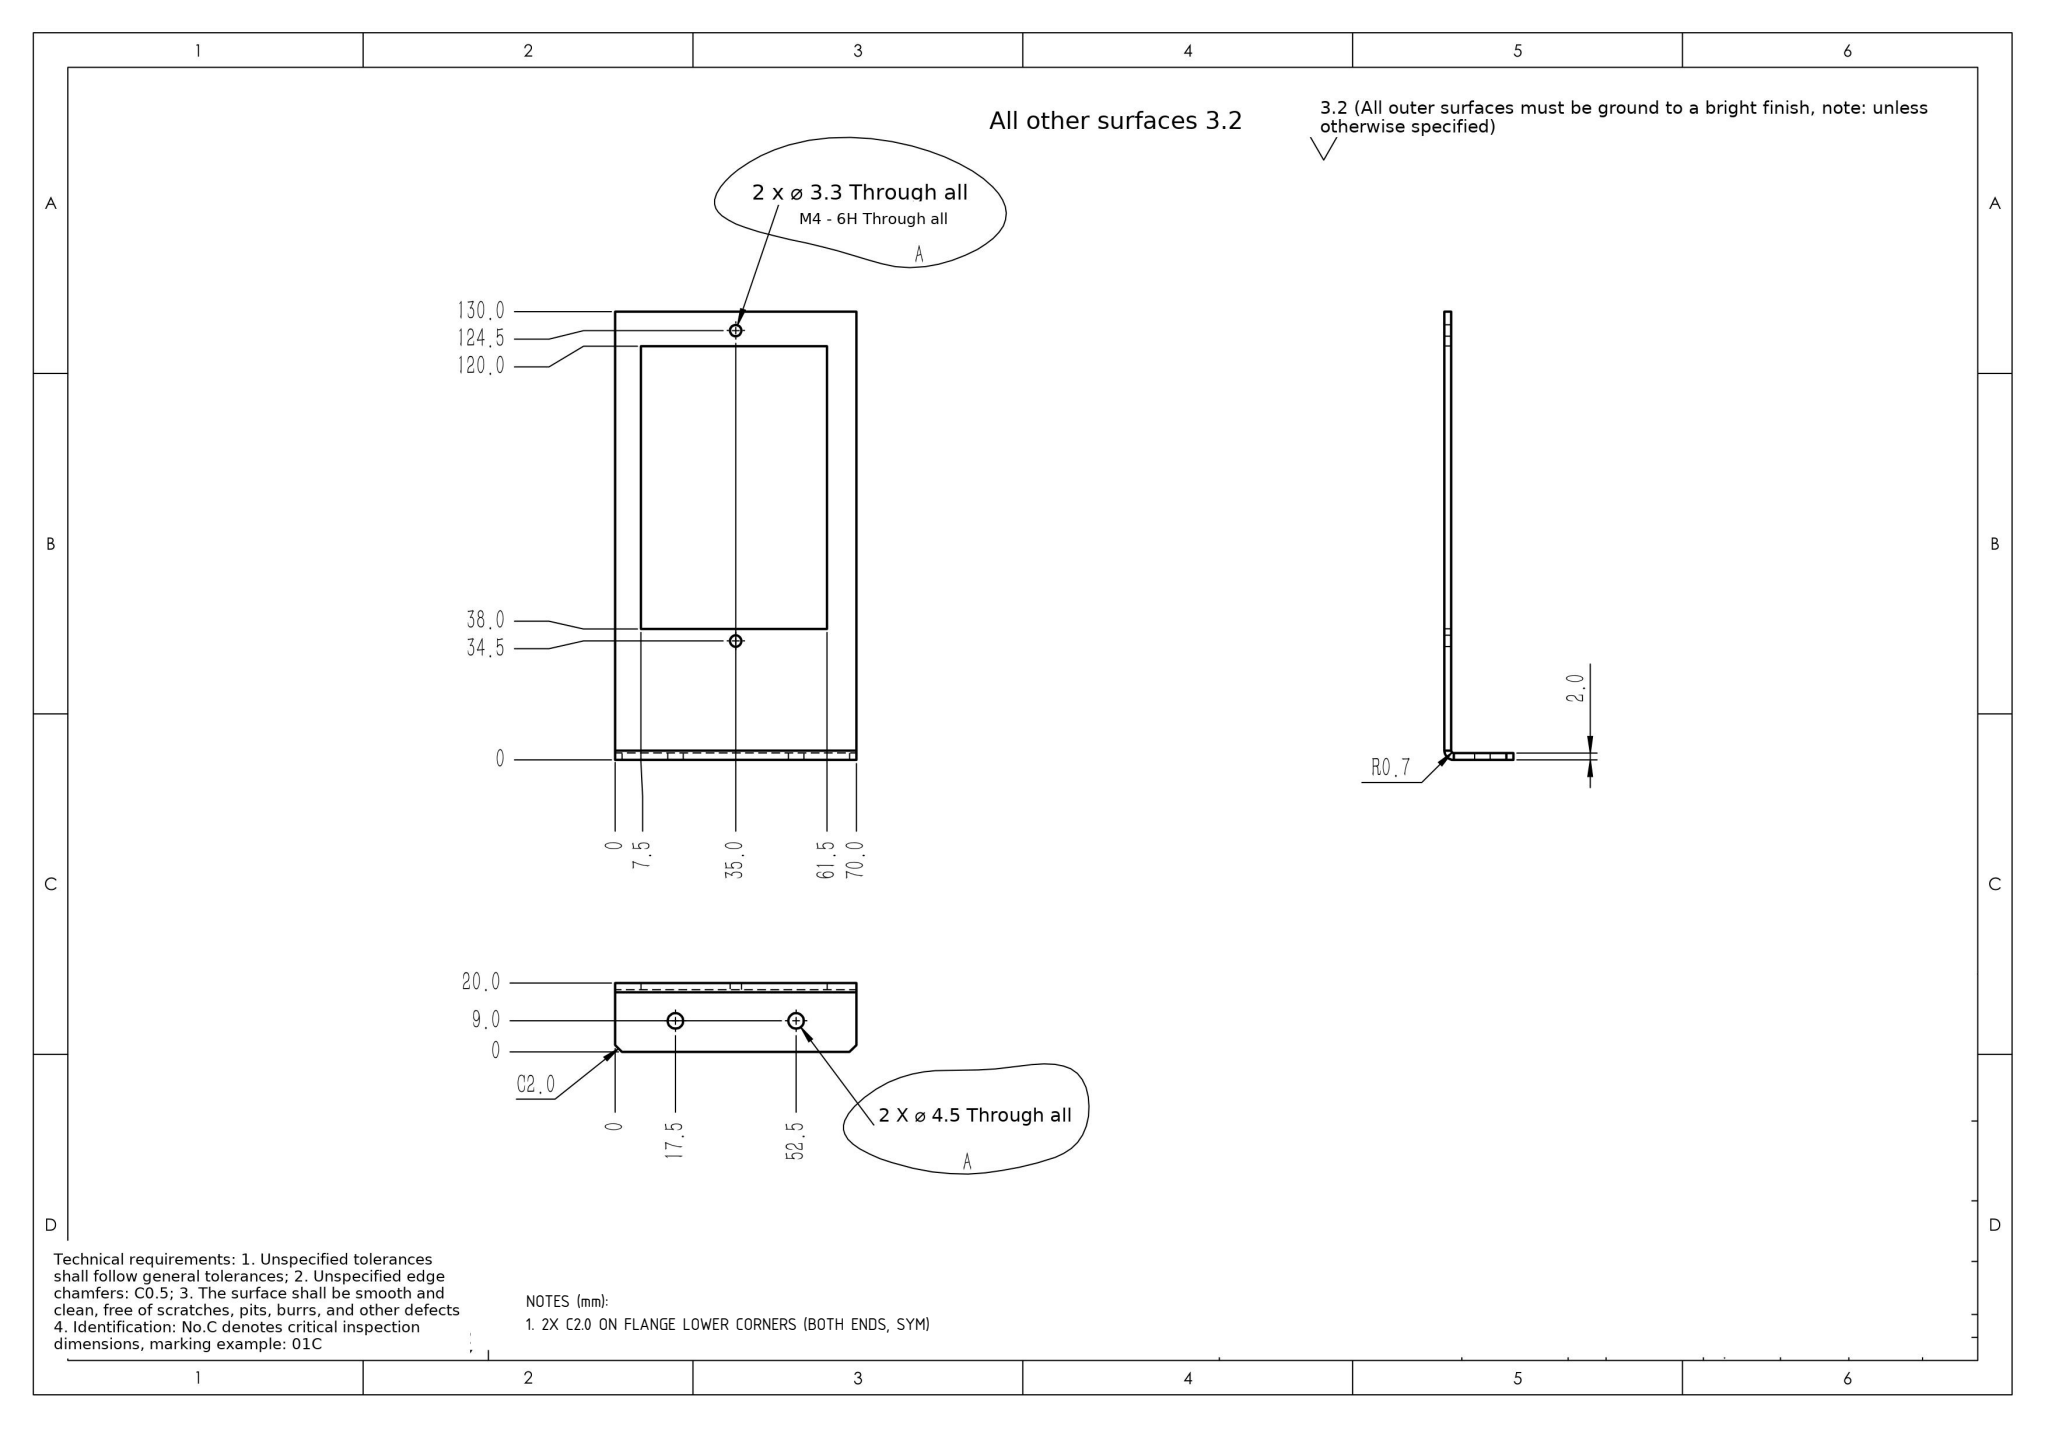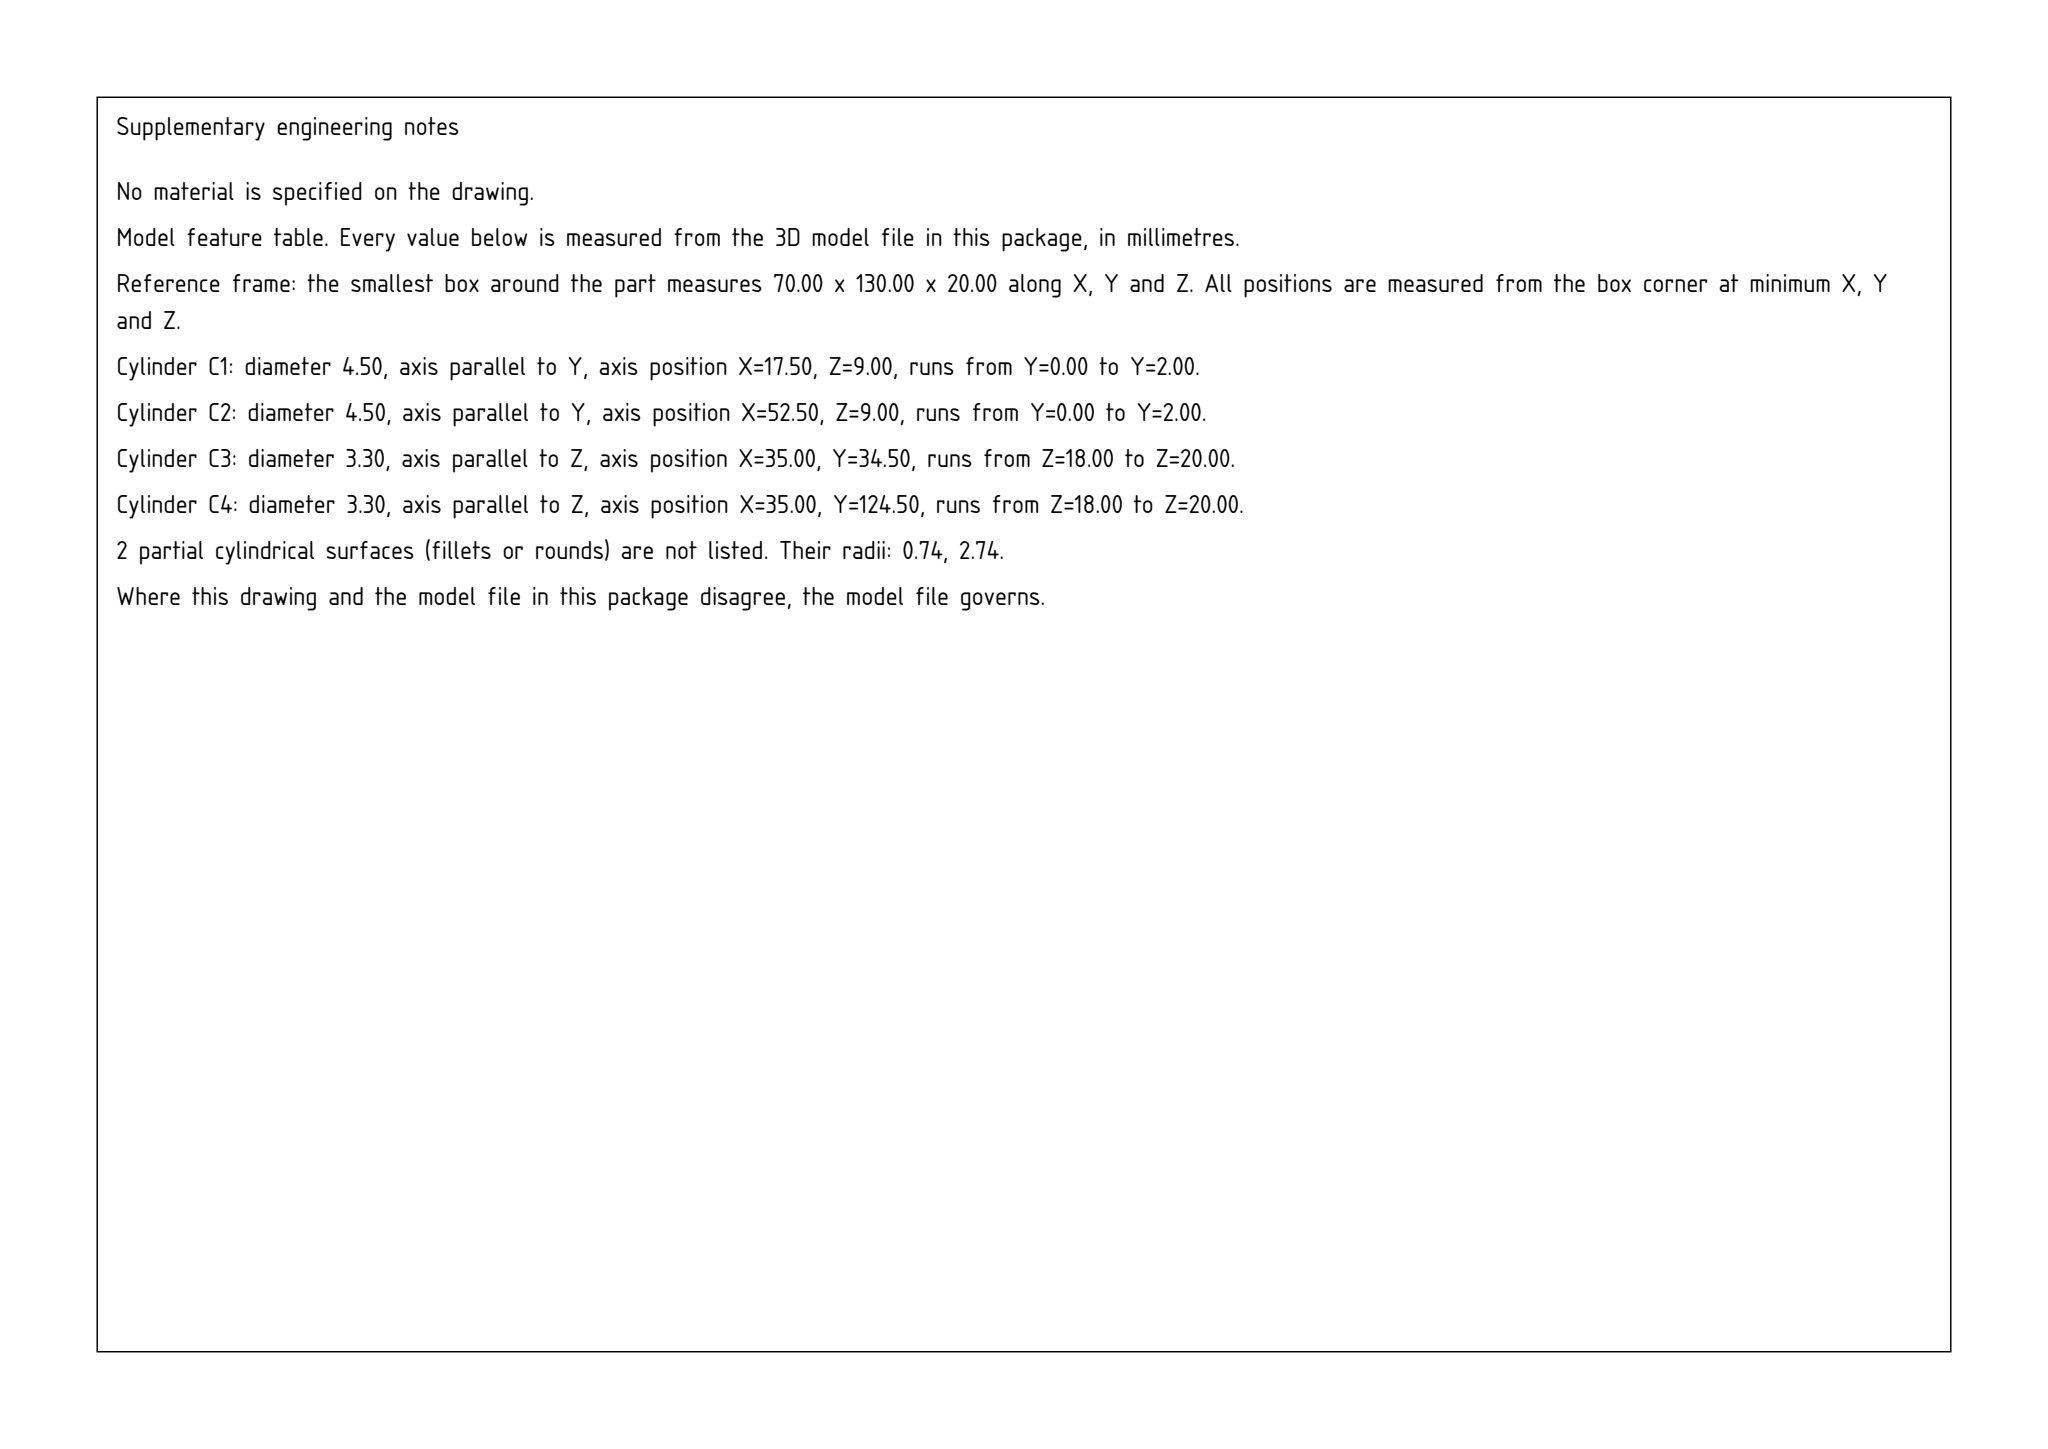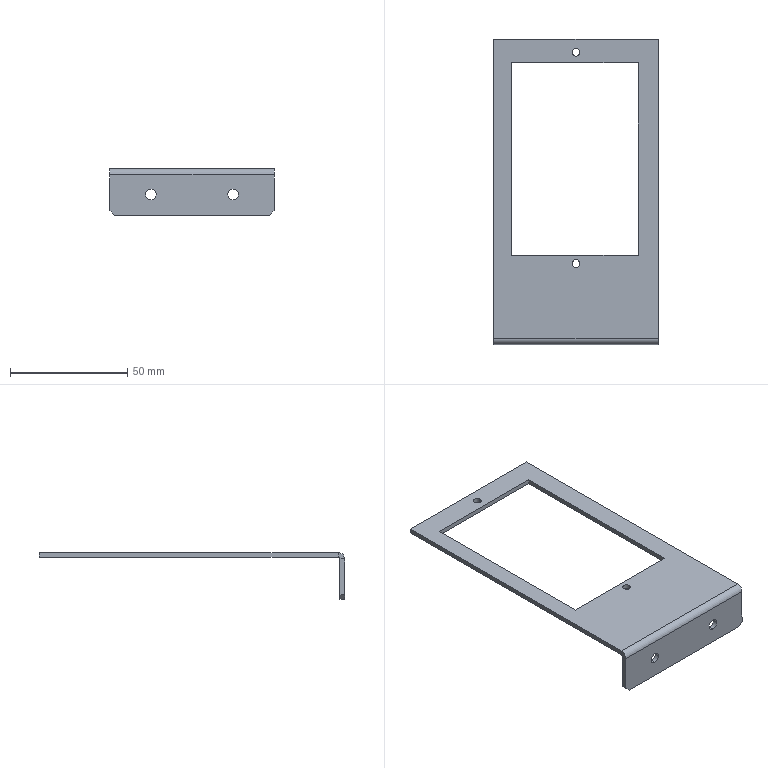Part | SolidWorks | mm | 1 solid | 28 faces | box 70 x 130 x 20 mm | volume 11654 mm3 | plane 18 | cylinder 10 | commonest cylinder face diameters 3.3 x4 4.5 x4 5.473 x1 1.473 x1
Drawing notes:
2X C2.0 ON FLANGE LOWER CORNERS (BOTH ENDS, SYM) | from the solid: x=0 and x=70 each have 3 planes incl. chamfer face; flange 70 long, z 0-20, chamfer 2x2 at both lower corners
STEP:
#1=CARTESIAN_POINT('',(36.65,34.5,0.));
#2=VERTEX_POINT('',#1);
#3=CARTESIAN_POINT('',(33.35,34.5,0.));
#4=VERTEX_POINT('',#3);
#5=CARTESIAN_POINT('',(35.,34.5,0.));
#6=DIRECTION('',(0.,0.,-1.));
#7=DIRECTION('',(-1.,0.,0.));
#8=AXIS2_PLACEMENT_3D('',#5,#6,#7);
#9=CIRCLE('',#8,1.65);
#10=EDGE_CURVE('',#2,#4,#9,.T.);
#11=ORIENTED_EDGE('',*,*,#10,.F.);
#12=CARTESIAN_POINT('',(36.65,34.5,-2.));
#13=VERTEX_POINT('',#12);
#14=CARTESIAN_POINT('',(36.65,34.5,-2.));
#15=DIRECTION('',(0.,0.,-1.));
#16=VECTOR('',#15,1000.);
#17=LINE('',#14,#16);
#18=EDGE_CURVE('',#2,#13,#17,.T.);
#19=ORIENTED_EDGE('',*,*,#18,.T.);
#20=CARTESIAN_POINT('',(33.35,34.5,-2.));
#21=VERTEX_POINT('',#20);
#22=CARTESIAN_POINT('',(35.,34.5,-2.));
#23=DIRECTION('',(0.,0.,-1.));
#24=DIRECTION('',(-1.,0.,0.));
#25=AXIS2_PLACEMENT_3D('',#22,#23,#24);
#26=CIRCLE('',#25,1.65);
#27=EDGE_CURVE('',#13,#21,#26,.T.);
#28=ORIENTED_EDGE('',*,*,#27,.T.);
#29=CARTESIAN_POINT('',(33.35,34.5,-2.));
#30=DIRECTION('',(0.,0.,-1.));
#31=VECTOR('',#30,1000.);
#32=LINE('',#29,#31);
#33=EDGE_CURVE('',#4,#21,#32,.T.);
#34=ORIENTED_EDGE('',*,*,#33,.F.);
#35=EDGE_LOOP('',(#11,#19,#28,#34));
#36=FACE_OUTER_BOUND('',#35,.T.);
#37=CARTESIAN_POINT('',(35.,34.5,-2.));
#38=DIRECTION('',(0.,0.,-1.));
#39=DIRECTION('',(-1.,0.,0.));
#40=AXIS2_PLACEMENT_3D('',#37,#38,#39);
#41=CYLINDRICAL_SURFACE('',#40,1.65);
#42=ADVANCED_FACE('',(#36),#41,.F.);
#43=CARTESIAN_POINT('',(36.65,124.5,0.));
#44=VERTEX_POINT('',#43);
#45=CARTESIAN_POINT('',(33.35,124.5,0.));
#46=VERTEX_POINT('',#45);
#47=CARTESIAN_POINT('',(35.,124.5,0.));
#48=DIRECTION('',(0.,0.,-1.));
#49=DIRECTION('',(-1.,0.,0.));
#50=AXIS2_PLACEMENT_3D('',#47,#48,#49);
#51=CIRCLE('',#50,1.65);
#52=EDGE_CURVE('',#44,#46,#51,.T.);
#53=ORIENTED_EDGE('',*,*,#52,.F.);
#54=CARTESIAN_POINT('',(36.65,124.5,-2.));
#55=VERTEX_POINT('',#54);
#56=CARTESIAN_POINT('',(36.65,124.5,-2.));
#57=DIRECTION('',(0.,0.,-1.));
#58=VECTOR('',#57,1000.);
#59=LINE('',#56,#58);
#60=EDGE_CURVE('',#44,#55,#59,.T.);
#61=ORIENTED_EDGE('',*,*,#60,.T.);
#62=CARTESIAN_POINT('',(33.35,124.5,-2.));
#63=VERTEX_POINT('',#62);
#64=CARTESIAN_POINT('',(35.,124.5,-2.));
#65=DIRECTION('',(0.,0.,-1.));
#66=DIRECTION('',(-1.,0.,0.));
#67=AXIS2_PLACEMENT_3D('',#64,#65,#66);
#68=CIRCLE('',#67,1.65);
#69=EDGE_CURVE('',#55,#63,#68,.T.);
#70=ORIENTED_EDGE('',*,*,#69,.T.);
#71=CARTESIAN_POINT('',(33.35,124.5,-2.));
#72=DIRECTION('',(0.,0.,-1.));
#73=VECTOR('',#72,1000.);
#74=LINE('',#71,#73);
#75=EDGE_CURVE('',#46,#63,#74,.T.);
#76=ORIENTED_EDGE('',*,*,#75,.F.);
#77=EDGE_LOOP('',(#53,#61,#70,#76));
#78=FACE_OUTER_BOUND('',#77,.T.);
#79=CARTESIAN_POINT('',(35.,124.5,-2.));
#80=DIRECTION('',(0.,0.,-1.));
#81=DIRECTION('',(-1.,0.,0.));
#82=AXIS2_PLACEMENT_3D('',#79,#80,#81);
#83=CYLINDRICAL_SURFACE('',#82,1.65);
#84=ADVANCED_FACE('',(#78),#83,.F.);
#85=CARTESIAN_POINT('',(52.5,-0.,-13.25));
#86=VERTEX_POINT('',#85);
#87=CARTESIAN_POINT('',(52.5,-0.,-8.75));
#88=VERTEX_POINT('',#87);
#89=CARTESIAN_POINT('',(52.5,-0.,-11.));
#90=DIRECTION('',(0.,1.,-0.));
#91=DIRECTION('',(0.,0.,1.));
#92=AXIS2_PLACEMENT_3D('',#89,#90,#91);
#93=CIRCLE('',#92,2.25);
#94=EDGE_CURVE('',#86,#88,#93,.T.);
#95=ORIENTED_EDGE('',*,*,#94,.F.);
#96=CARTESIAN_POINT('',(52.5,2.,-13.25));
#97=VERTEX_POINT('',#96);
#98=CARTESIAN_POINT('',(52.5,2.,-13.25));
#99=DIRECTION('',(0.,1.,-0.));
#100=VECTOR('',#99,1000.);
#101=LINE('',#98,#100);
#102=EDGE_CURVE('',#86,#97,#101,.T.);
#103=ORIENTED_EDGE('',*,*,#102,.T.);
#104=CARTESIAN_POINT('',(52.5,2.,-8.75));
#105=VERTEX_POINT('',#104);
#106=CARTESIAN_POINT('',(52.5,2.,-11.));
#107=DIRECTION('',(0.,1.,-0.));
#108=DIRECTION('',(0.,0.,1.));
#109=AXIS2_PLACEMENT_3D('',#106,#107,#108);
#110=CIRCLE('',#109,2.25);
#111=EDGE_CURVE('',#97,#105,#110,.T.);
#112=ORIENTED_EDGE('',*,*,#111,.T.);
#113=CARTESIAN_POINT('',(52.5,2.,-8.75));
#114=DIRECTION('',(0.,1.,-0.));
#115=VECTOR('',#114,1000.);
#116=LINE('',#113,#115);
#117=EDGE_CURVE('',#88,#105,#116,.T.);
#118=ORIENTED_EDGE('',*,*,#117,.F.);
#119=EDGE_LOOP('',(#95,#103,#112,#118));
#120=FACE_OUTER_BOUND('',#119,.T.);
#121=CARTESIAN_POINT('',(52.5,2.,-11.));
#122=DIRECTION('',(0.,1.,-0.));
#123=DIRECTION('',(0.,0.,1.));
#124=AXIS2_PLACEMENT_3D('',#121,#122,#123);
#125=CYLINDRICAL_SURFACE('',#124,2.25);
#126=ADVANCED_FACE('',(#120),#125,.F.);
#127=CARTESIAN_POINT('',(17.5,-0.,-13.25));
#128=VERTEX_POINT('',#127);
#129=CARTESIAN_POINT('',(17.5,-0.,-8.75));
#130=VERTEX_POINT('',#129);
#131=CARTESIAN_POINT('',(17.5,-0.,-11.));
#132=DIRECTION('',(0.,1.,-0.));
#133=DIRECTION('',(0.,0.,1.));
#134=AXIS2_PLACEMENT_3D('',#131,#132,#133);
#135=CIRCLE('',#134,2.25);
#136=EDGE_CURVE('',#128,#130,#135,.T.);
#137=ORIENTED_EDGE('',*,*,#136,.F.);
#138=CARTESIAN_POINT('',(17.5,2.,-13.25));
#139=VERTEX_POINT('',#138);
#140=CARTESIAN_POINT('',(17.5,2.,-13.25));
#141=DIRECTION('',(0.,1.,-0.));
#142=VECTOR('',#141,1000.);
#143=LINE('',#140,#142);
#144=EDGE_CURVE('',#128,#139,#143,.T.);
#145=ORIENTED_EDGE('',*,*,#144,.T.);
#146=CARTESIAN_POINT('',(17.5,2.,-8.75));
#147=VERTEX_POINT('',#146);
#148=CARTESIAN_POINT('',(17.5,2.,-11.));
#149=DIRECTION('',(0.,1.,-0.));
#150=DIRECTION('',(0.,0.,1.));
#151=AXIS2_PLACEMENT_3D('',#148,#149,#150);
#152=CIRCLE('',#151,2.25);
#153=EDGE_CURVE('',#139,#147,#152,.T.);
#154=ORIENTED_EDGE('',*,*,#153,.T.);
#155=CARTESIAN_POINT('',(17.5,2.,-8.75));
#156=DIRECTION('',(0.,1.,-0.));
#157=VECTOR('',#156,1000.);
#158=LINE('',#155,#157);
#159=EDGE_CURVE('',#130,#147,#158,.T.);
#160=ORIENTED_EDGE('',*,*,#159,.F.);
#161=EDGE_LOOP('',(#137,#145,#154,#160));
#162=FACE_OUTER_BOUND('',#161,.T.);
#163=CARTESIAN_POINT('',(17.5,2.,-11.));
#164=DIRECTION('',(0.,1.,-0.));
#165=DIRECTION('',(0.,0.,1.));
#166=AXIS2_PLACEMENT_3D('',#163,#164,#165);
#167=CYLINDRICAL_SURFACE('',#166,2.25);
#168=ADVANCED_FACE('',(#162),#167,.F.);
#169=CARTESIAN_POINT('',(0.,130.,-2.));
#170=VERTEX_POINT('',#169);
#171=CARTESIAN_POINT('',(0.,2.737,-2.));
#172=VERTEX_POINT('',#171);
#173=CARTESIAN_POINT('',(0.,0.,-2.));
#174=DIRECTION('',(0.,-1.,0.));
#175=VECTOR('',#174,1000.);
#176=LINE('',#173,#175);
#177=EDGE_CURVE('',#170,#172,#176,.T.);
#178=ORIENTED_EDGE('',*,*,#177,.T.);
#179=CARTESIAN_POINT('',(0.,2.737,-0.));
#180=VERTEX_POINT('',#179);
#181=CARTESIAN_POINT('',(0.,2.737,-2.));
#182=DIRECTION('',(-0.,0.,1.));
#183=VECTOR('',#182,1000.);
#184=LINE('',#181,#183);
#185=EDGE_CURVE('',#172,#180,#184,.T.);
#186=ORIENTED_EDGE('',*,*,#185,.T.);
#187=CARTESIAN_POINT('',(0.,130.,0.));
#188=VERTEX_POINT('',#187);
#189=CARTESIAN_POINT('',(0.,0.,0.));
#190=DIRECTION('',(0.,-1.,0.));
#191=VECTOR('',#190,1000.);
#192=LINE('',#189,#191);
#193=EDGE_CURVE('',#188,#180,#192,.T.);
#194=ORIENTED_EDGE('',*,*,#193,.F.);
#195=CARTESIAN_POINT('',(0.,130.,-2.));
#196=DIRECTION('',(0.,0.,1.));
#197=VECTOR('',#196,1000.);
#198=LINE('',#195,#197);
#199=EDGE_CURVE('',#170,#188,#198,.T.);
#200=ORIENTED_EDGE('',*,*,#199,.F.);
#201=EDGE_LOOP('',(#178,#186,#194,#200));
#202=FACE_OUTER_BOUND('',#201,.T.);
#203=CARTESIAN_POINT('',(0.,0.,-2.));
#204=DIRECTION('',(-1.,0.,0.));
#205=DIRECTION('',(0.,0.,1.));
#206=AXIS2_PLACEMENT_3D('',#203,#204,#205);
#207=PLANE('',#206);
#208=ADVANCED_FACE('',(#202),#207,.T.);
#209=CARTESIAN_POINT('',(35.,34.5,-2.));
#210=DIRECTION('',(0.,0.,-1.));
#211=DIRECTION('',(-1.,0.,0.));
#212=AXIS2_PLACEMENT_3D('',#209,#210,#211);
#213=CIRCLE('',#212,1.65);
#214=EDGE_CURVE('',#21,#13,#213,.T.);
#215=ORIENTED_EDGE('',*,*,#214,.F.);
#216=ORIENTED_EDGE('',*,*,#27,.F.);
#217=EDGE_LOOP('',(#215,#216));
#218=FACE_BOUND('',#217,.T.);
#219=CARTESIAN_POINT('',(35.,124.5,-2.));
#220=DIRECTION('',(0.,0.,-1.));
#221=DIRECTION('',(-1.,0.,0.));
#222=AXIS2_PLACEMENT_3D('',#219,#220,#221);
#223=CIRCLE('',#222,1.65);
#224=EDGE_CURVE('',#63,#55,#223,.T.);
#225=ORIENTED_EDGE('',*,*,#224,.F.);
#226=ORIENTED_EDGE('',*,*,#69,.F.);
#227=EDGE_LOOP('',(#225,#226));
#228=FACE_BOUND('',#227,.T.);
#229=CARTESIAN_POINT('',(7.5,38.,-2.));
#230=VERTEX_POINT('',#229);
#231=CARTESIAN_POINT('',(7.5,120.,-2.));
#232=VERTEX_POINT('',#231);
#233=CARTESIAN_POINT('',(7.5,120.,-2.));
#234=DIRECTION('',(0.,1.,0.));
#235=VECTOR('',#234,1000.);
#236=LINE('',#233,#235);
#237=EDGE_CURVE('',#230,#232,#236,.T.);
#238=ORIENTED_EDGE('',*,*,#237,.F.);
#239=CARTESIAN_POINT('',(61.5,38.,-2.));
#240=VERTEX_POINT('',#239);
#241=CARTESIAN_POINT('',(7.5,38.,-2.));
#242=DIRECTION('',(-1.,0.,0.));
#243=VECTOR('',#242,1000.);
#244=LINE('',#241,#243);
#245=EDGE_CURVE('',#240,#230,#244,.T.);
#246=ORIENTED_EDGE('',*,*,#245,.F.);
#247=CARTESIAN_POINT('',(61.5,120.,-2.));
#248=VERTEX_POINT('',#247);
#249=CARTESIAN_POINT('',(61.5,120.,-2.));
#250=DIRECTION('',(0.,-1.,0.));
#251=VECTOR('',#250,1000.);
#252=LINE('',#249,#251);
#253=EDGE_CURVE('',#248,#240,#252,.T.);
#254=ORIENTED_EDGE('',*,*,#253,.F.);
#255=CARTESIAN_POINT('',(7.5,120.,-2.));
#256=DIRECTION('',(1.,0.,0.));
#257=VECTOR('',#256,1000.);
#258=LINE('',#255,#257);
#259=EDGE_CURVE('',#232,#248,#258,.T.);
#260=ORIENTED_EDGE('',*,*,#259,.F.);
#261=EDGE_LOOP('',(#238,#246,#254,#260));
#262=FACE_BOUND('',#261,.T.);
#263=CARTESIAN_POINT('',(70.,2.737,-2.));
#264=VERTEX_POINT('',#263);
#265=CARTESIAN_POINT('',(70.,130.,-2.));
#266=VERTEX_POINT('',#265);
#267=CARTESIAN_POINT('',(70.,0.,-2.));
#268=DIRECTION('',(0.,1.,0.));
#269=VECTOR('',#268,1000.);
#270=LINE('',#267,#269);
#271=EDGE_CURVE('',#264,#266,#270,.T.);
#272=ORIENTED_EDGE('',*,*,#271,.F.);
#273=CARTESIAN_POINT('',(0.,2.737,-2.));
#274=DIRECTION('',(1.,0.,0.));
#275=VECTOR('',#274,1000.);
#276=LINE('',#273,#275);
#277=EDGE_CURVE('',#172,#264,#276,.T.);
#278=ORIENTED_EDGE('',*,*,#277,.F.);
#279=ORIENTED_EDGE('',*,*,#177,.F.);
#280=CARTESIAN_POINT('',(0.,130.,-2.));
#281=DIRECTION('',(-1.,0.,0.));
#282=VECTOR('',#281,1000.);
#283=LINE('',#280,#282);
#284=EDGE_CURVE('',#266,#170,#283,.T.);
#285=ORIENTED_EDGE('',*,*,#284,.F.);
#286=EDGE_LOOP('',(#272,#278,#279,#285));
#287=FACE_OUTER_BOUND('',#286,.T.);
#288=CARTESIAN_POINT('',(0.,0.,-2.));
#289=DIRECTION('',(0.,0.,-1.));
#290=DIRECTION('',(-1.,0.,0.));
#291=AXIS2_PLACEMENT_3D('',#288,#289,#290);
#292=PLANE('',#291);
#293=ADVANCED_FACE('',(#218,#228,#262,#287),#292,.T.);
#294=CARTESIAN_POINT('',(35.,34.5,0.));
#295=DIRECTION('',(0.,0.,-1.));
#296=DIRECTION('',(-1.,0.,0.));
#297=AXIS2_PLACEMENT_3D('',#294,#295,#296);
#298=CIRCLE('',#297,1.65);
#299=EDGE_CURVE('',#4,#2,#298,.T.);
#300=ORIENTED_EDGE('',*,*,#299,.T.);
#301=ORIENTED_EDGE('',*,*,#10,.T.);
#302=EDGE_LOOP('',(#300,#301));
#303=FACE_BOUND('',#302,.T.);
#304=CARTESIAN_POINT('',(35.,124.5,0.));
#305=DIRECTION('',(0.,0.,-1.));
#306=DIRECTION('',(-1.,0.,0.));
#307=AXIS2_PLACEMENT_3D('',#304,#305,#306);
#308=CIRCLE('',#307,1.65);
#309=EDGE_CURVE('',#46,#44,#308,.T.);
#310=ORIENTED_EDGE('',*,*,#309,.T.);
#311=ORIENTED_EDGE('',*,*,#52,.T.);
#312=EDGE_LOOP('',(#310,#311));
#313=FACE_BOUND('',#312,.T.);
#314=CARTESIAN_POINT('',(61.5,38.,0.));
#315=VERTEX_POINT('',#314);
#316=CARTESIAN_POINT('',(7.5,38.,0.));
#317=VERTEX_POINT('',#316);
#318=CARTESIAN_POINT('',(0.,38.,0.));
#319=DIRECTION('',(-1.,0.,0.));
#320=VECTOR('',#319,1000.);
#321=LINE('',#318,#320);
#322=EDGE_CURVE('',#315,#317,#321,.T.);
#323=ORIENTED_EDGE('',*,*,#322,.T.);
#324=CARTESIAN_POINT('',(7.5,120.,0.));
#325=VERTEX_POINT('',#324);
#326=CARTESIAN_POINT('',(7.5,-0.,0.));
#327=DIRECTION('',(0.,1.,0.));
#328=VECTOR('',#327,1000.);
#329=LINE('',#326,#328);
#330=EDGE_CURVE('',#317,#325,#329,.T.);
#331=ORIENTED_EDGE('',*,*,#330,.T.);
#332=CARTESIAN_POINT('',(61.5,120.,0.));
#333=VERTEX_POINT('',#332);
#334=CARTESIAN_POINT('',(0.,120.,0.));
#335=DIRECTION('',(1.,0.,0.));
#336=VECTOR('',#335,1000.);
#337=LINE('',#334,#336);
#338=EDGE_CURVE('',#325,#333,#337,.T.);
#339=ORIENTED_EDGE('',*,*,#338,.T.);
#340=CARTESIAN_POINT('',(61.5,0.,0.));
#341=DIRECTION('',(0.,-1.,0.));
#342=VECTOR('',#341,1000.);
#343=LINE('',#340,#342);
#344=EDGE_CURVE('',#333,#315,#343,.T.);
#345=ORIENTED_EDGE('',*,*,#344,.T.);
#346=EDGE_LOOP('',(#323,#331,#339,#345));
#347=FACE_BOUND('',#346,.T.);
#348=CARTESIAN_POINT('',(70.,2.737,0.));
#349=VERTEX_POINT('',#348);
#350=CARTESIAN_POINT('',(0.,2.737,-0.));
#351=DIRECTION('',(1.,0.,0.));
#352=VECTOR('',#351,1000.);
#353=LINE('',#350,#352);
#354=EDGE_CURVE('',#180,#349,#353,.T.);
#355=ORIENTED_EDGE('',*,*,#354,.T.);
#356=CARTESIAN_POINT('',(70.,130.,0.));
#357=VERTEX_POINT('',#356);
#358=CARTESIAN_POINT('',(70.,0.,0.));
#359=DIRECTION('',(0.,1.,0.));
#360=VECTOR('',#359,1000.);
#361=LINE('',#358,#360);
#362=EDGE_CURVE('',#349,#357,#361,.T.);
#363=ORIENTED_EDGE('',*,*,#362,.T.);
#364=CARTESIAN_POINT('',(0.,130.,0.));
#365=DIRECTION('',(-1.,0.,0.));
#366=VECTOR('',#365,1000.);
#367=LINE('',#364,#366);
#368=EDGE_CURVE('',#357,#188,#367,.T.);
#369=ORIENTED_EDGE('',*,*,#368,.T.);
#370=ORIENTED_EDGE('',*,*,#193,.T.);
#371=EDGE_LOOP('',(#355,#363,#369,#370));
#372=FACE_OUTER_BOUND('',#371,.T.);
#373=CARTESIAN_POINT('',(0.,0.,0.));
#374=DIRECTION('',(0.,0.,-1.));
#375=DIRECTION('',(-1.,0.,0.));
#376=AXIS2_PLACEMENT_3D('',#373,#374,#375);
#377=PLANE('',#376);
#378=ADVANCED_FACE('',(#303,#313,#347,#372),#377,.F.);
#379=ORIENTED_EDGE('',*,*,#368,.F.);
#380=CARTESIAN_POINT('',(70.,130.,-2.));
#381=DIRECTION('',(0.,0.,1.));
#382=VECTOR('',#381,1000.);
#383=LINE('',#380,#382);
#384=EDGE_CURVE('',#266,#357,#383,.T.);
#385=ORIENTED_EDGE('',*,*,#384,.F.);
#386=ORIENTED_EDGE('',*,*,#284,.T.);
#387=ORIENTED_EDGE('',*,*,#199,.T.);
#388=EDGE_LOOP('',(#379,#385,#386,#387));
#389=FACE_OUTER_BOUND('',#388,.T.);
#390=CARTESIAN_POINT('',(0.,130.,-2.));
#391=DIRECTION('',(0.,1.,0.));
#392=DIRECTION('',(0.,0.,1.));
#393=AXIS2_PLACEMENT_3D('',#390,#391,#392);
#394=PLANE('',#393);
#395=ADVANCED_FACE('',(#389),#394,.T.);
#396=CARTESIAN_POINT('',(70.,2.737,-2.));
#397=DIRECTION('',(0.,0.,1.));
#398=VECTOR('',#397,1000.);
#399=LINE('',#396,#398);
#400=EDGE_CURVE('',#264,#349,#399,.T.);
#401=ORIENTED_EDGE('',*,*,#400,.F.);
#402=ORIENTED_EDGE('',*,*,#271,.T.);
#403=ORIENTED_EDGE('',*,*,#384,.T.);
#404=ORIENTED_EDGE('',*,*,#362,.F.);
#405=EDGE_LOOP('',(#401,#402,#403,#404));
#406=FACE_OUTER_BOUND('',#405,.T.);
#407=CARTESIAN_POINT('',(70.,0.,-2.));
#408=DIRECTION('',(1.,0.,0.));
#409=DIRECTION('',(0.,0.,-1.));
#410=AXIS2_PLACEMENT_3D('',#407,#408,#409);
#411=PLANE('',#410);
#412=ADVANCED_FACE('',(#406),#411,.T.);
#413=CARTESIAN_POINT('',(70.,2.,-2.737));
#414=VERTEX_POINT('',#413);
#415=CARTESIAN_POINT('',(70.,-0.,-2.737));
#416=VERTEX_POINT('',#415);
#417=CARTESIAN_POINT('',(70.,-0.,-2.737));
#418=DIRECTION('',(0.,-1.,0.));
#419=VECTOR('',#418,1000.);
#420=LINE('',#417,#419);
#421=EDGE_CURVE('',#414,#416,#420,.T.);
#422=ORIENTED_EDGE('',*,*,#421,.F.);
#423=CARTESIAN_POINT('',(70.,2.737,-2.737));
#424=DIRECTION('',(1.,0.,0.));
#425=DIRECTION('',(0.,0.,1.));
#426=AXIS2_PLACEMENT_3D('',#423,#424,#425);
#427=CIRCLE('',#426,0.7366);
#428=EDGE_CURVE('',#264,#414,#427,.T.);
#429=ORIENTED_EDGE('',*,*,#428,.F.);
#430=ORIENTED_EDGE('',*,*,#400,.T.);
#431=CARTESIAN_POINT('',(70.,2.737,-2.737));
#432=DIRECTION('',(1.,0.,0.));
#433=DIRECTION('',(0.,0.,1.));
#434=AXIS2_PLACEMENT_3D('',#431,#432,#433);
#435=CIRCLE('',#434,2.737);
#436=EDGE_CURVE('',#349,#416,#435,.T.);
#437=ORIENTED_EDGE('',*,*,#436,.T.);
#438=EDGE_LOOP('',(#422,#429,#430,#437));
#439=FACE_OUTER_BOUND('',#438,.T.);
#440=CARTESIAN_POINT('',(70.,2.737,-2.737));
#441=DIRECTION('',(1.,0.,0.));
#442=DIRECTION('',(0.,0.,-1.));
#443=AXIS2_PLACEMENT_3D('',#440,#441,#442);
#444=PLANE('',#443);
#445=ADVANCED_FACE('',(#439),#444,.T.);
#446=CARTESIAN_POINT('',(0.,2.,-2.737));
#447=VERTEX_POINT('',#446);
#448=CARTESIAN_POINT('',(0.,2.737,-2.737));
#449=DIRECTION('',(-1.,0.,0.));
#450=DIRECTION('',(0.,0.,1.));
#451=AXIS2_PLACEMENT_3D('',#448,#449,#450);
#452=CIRCLE('',#451,0.7366);
#453=EDGE_CURVE('',#447,#172,#452,.T.);
#454=ORIENTED_EDGE('',*,*,#453,.F.);
#455=CARTESIAN_POINT('',(0.,-0.,-2.737));
#456=VERTEX_POINT('',#455);
#457=CARTESIAN_POINT('',(0.,2.,-2.737));
#458=DIRECTION('',(0.,-1.,0.));
#459=VECTOR('',#458,1000.);
#460=LINE('',#457,#459);
#461=EDGE_CURVE('',#447,#456,#460,.T.);
#462=ORIENTED_EDGE('',*,*,#461,.T.);
#463=CARTESIAN_POINT('',(0.,2.737,-2.737));
#464=DIRECTION('',(-1.,0.,0.));
#465=DIRECTION('',(0.,0.,1.));
#466=AXIS2_PLACEMENT_3D('',#463,#464,#465);
#467=CIRCLE('',#466,2.737);
#468=EDGE_CURVE('',#456,#180,#467,.T.);
#469=ORIENTED_EDGE('',*,*,#468,.T.);
#470=ORIENTED_EDGE('',*,*,#185,.F.);
#471=EDGE_LOOP('',(#454,#462,#469,#470));
#472=FACE_OUTER_BOUND('',#471,.T.);
#473=CARTESIAN_POINT('',(0.,2.737,-2.737));
#474=DIRECTION('',(1.,0.,0.));
#475=DIRECTION('',(0.,0.,-1.));
#476=AXIS2_PLACEMENT_3D('',#473,#474,#475);
#477=PLANE('',#476);
#478=ADVANCED_FACE('',(#472),#477,.F.);
#479=ORIENTED_EDGE('',*,*,#354,.F.);
#480=ORIENTED_EDGE('',*,*,#468,.F.);
#481=CARTESIAN_POINT('',(70.,-0.,-2.737));
#482=DIRECTION('',(1.,0.,0.));
#483=VECTOR('',#482,1000.);
#484=LINE('',#481,#483);
#485=EDGE_CURVE('',#456,#416,#484,.T.);
#486=ORIENTED_EDGE('',*,*,#485,.T.);
#487=ORIENTED_EDGE('',*,*,#436,.F.);
#488=EDGE_LOOP('',(#479,#480,#486,#487));
#489=FACE_OUTER_BOUND('',#488,.T.);
#490=CARTESIAN_POINT('',(0.,2.737,-2.737));
#491=DIRECTION('',(-1.,0.,0.));
#492=DIRECTION('',(0.,-1.,0.));
#493=AXIS2_PLACEMENT_3D('',#490,#491,#492);
#494=CYLINDRICAL_SURFACE('',#493,2.737);
#495=ADVANCED_FACE('',(#489),#494,.T.);
#496=ORIENTED_EDGE('',*,*,#277,.T.);
#497=ORIENTED_EDGE('',*,*,#428,.T.);
#498=CARTESIAN_POINT('',(70.,2.,-2.737));
#499=DIRECTION('',(-1.,0.,0.));
#500=VECTOR('',#499,1000.);
#501=LINE('',#498,#500);
#502=EDGE_CURVE('',#414,#447,#501,.T.);
#503=ORIENTED_EDGE('',*,*,#502,.T.);
#504=ORIENTED_EDGE('',*,*,#453,.T.);
#505=EDGE_LOOP('',(#496,#497,#503,#504));
#506=FACE_OUTER_BOUND('',#505,.T.);
#507=CARTESIAN_POINT('',(0.,2.737,-2.737));
#508=DIRECTION('',(-1.,0.,0.));
#509=DIRECTION('',(0.,-1.,0.));
#510=AXIS2_PLACEMENT_3D('',#507,#508,#509);
#511=CYLINDRICAL_SURFACE('',#510,0.7366);
#512=ADVANCED_FACE('',(#506),#511,.F.);
#513=CARTESIAN_POINT('',(0.,2.,-18.));
#514=VERTEX_POINT('',#513);
#515=CARTESIAN_POINT('',(0.,2.,-20.));
#516=DIRECTION('',(0.,-0.,-1.));
#517=VECTOR('',#516,1000.);
#518=LINE('',#515,#517);
#519=EDGE_CURVE('',#447,#514,#518,.T.);
#520=ORIENTED_EDGE('',*,*,#519,.T.);
#521=CARTESIAN_POINT('',(-0.,-0.,-18.));
#522=VERTEX_POINT('',#521);
#523=CARTESIAN_POINT('',(0.,-0.,-18.));
#524=DIRECTION('',(0.,-1.,0.));
#525=VECTOR('',#524,1000.);
#526=LINE('',#523,#525);
#527=EDGE_CURVE('',#514,#522,#526,.T.);
#528=ORIENTED_EDGE('',*,*,#527,.T.);
#529=CARTESIAN_POINT('',(0.,0.,0.));
#530=DIRECTION('',(0.,-0.,-1.));
#531=VECTOR('',#530,1000.);
#532=LINE('',#529,#531);
#533=EDGE_CURVE('',#456,#522,#532,.T.);
#534=ORIENTED_EDGE('',*,*,#533,.F.);
#535=ORIENTED_EDGE('',*,*,#461,.F.);
#536=EDGE_LOOP('',(#520,#528,#534,#535));
#537=FACE_OUTER_BOUND('',#536,.T.);
#538=CARTESIAN_POINT('',(0.,-0.,-20.));
#539=DIRECTION('',(1.,0.,0.));
#540=DIRECTION('',(0.,0.,-1.));
#541=AXIS2_PLACEMENT_3D('',#538,#539,#540);
#542=PLANE('',#541);
#543=ADVANCED_FACE('',(#537),#542,.F.);
#544=CARTESIAN_POINT('',(70.,-0.,-18.));
#545=VERTEX_POINT('',#544);
#546=CARTESIAN_POINT('',(70.,0.,0.));
#547=DIRECTION('',(0.,0.,1.));
#548=VECTOR('',#547,1000.);
#549=LINE('',#546,#548);
#550=EDGE_CURVE('',#545,#416,#549,.T.);
#551=ORIENTED_EDGE('',*,*,#550,.F.);
#552=CARTESIAN_POINT('',(70.,2.,-18.));
#553=VERTEX_POINT('',#552);
#554=CARTESIAN_POINT('',(70.,-0.,-18.));
#555=DIRECTION('',(0.,1.,-0.));
#556=VECTOR('',#555,1000.);
#557=LINE('',#554,#556);
#558=EDGE_CURVE('',#545,#553,#557,.T.);
#559=ORIENTED_EDGE('',*,*,#558,.T.);
#560=CARTESIAN_POINT('',(70.,2.,-2.));
#561=DIRECTION('',(0.,0.,1.));
#562=VECTOR('',#561,1000.);
#563=LINE('',#560,#562);
#564=EDGE_CURVE('',#553,#414,#563,.T.);
#565=ORIENTED_EDGE('',*,*,#564,.T.);
#566=ORIENTED_EDGE('',*,*,#421,.T.);
#567=EDGE_LOOP('',(#551,#559,#565,#566));
#568=FACE_OUTER_BOUND('',#567,.T.);
#569=CARTESIAN_POINT('',(70.,0.,-2.));
#570=DIRECTION('',(-1.,0.,0.));
#571=DIRECTION('',(0.,0.,1.));
#572=AXIS2_PLACEMENT_3D('',#569,#570,#571);
#573=PLANE('',#572);
#574=ADVANCED_FACE('',(#568),#573,.F.);
#575=CARTESIAN_POINT('',(52.5,-0.,-11.));
#576=DIRECTION('',(0.,1.,-0.));
#577=DIRECTION('',(0.,0.,1.));
#578=AXIS2_PLACEMENT_3D('',#575,#576,#577);
#579=CIRCLE('',#578,2.25);
#580=EDGE_CURVE('',#88,#86,#579,.T.);
#581=ORIENTED_EDGE('',*,*,#580,.T.);
#582=ORIENTED_EDGE('',*,*,#94,.T.);
#583=EDGE_LOOP('',(#581,#582));
#584=FACE_BOUND('',#583,.T.);
#585=CARTESIAN_POINT('',(17.5,-0.,-11.));
#586=DIRECTION('',(0.,1.,-0.));
#587=DIRECTION('',(0.,0.,1.));
#588=AXIS2_PLACEMENT_3D('',#585,#586,#587);
#589=CIRCLE('',#588,2.25);
#590=EDGE_CURVE('',#130,#128,#589,.T.);
#591=ORIENTED_EDGE('',*,*,#590,.T.);
#592=ORIENTED_EDGE('',*,*,#136,.T.);
#593=EDGE_LOOP('',(#591,#592));
#594=FACE_BOUND('',#593,.T.);
#595=ORIENTED_EDGE('',*,*,#533,.T.);
#596=CARTESIAN_POINT('',(2.,-0.,-20.));
#597=VERTEX_POINT('',#596);
#598=CARTESIAN_POINT('',(2.,-0.,-20.));
#599=DIRECTION('',(0.7071,-0.,-0.7071));
#600=VECTOR('',#599,1000.);
#601=LINE('',#598,#600);
#602=EDGE_CURVE('',#522,#597,#601,.T.);
#603=ORIENTED_EDGE('',*,*,#602,.T.);
#604=CARTESIAN_POINT('',(68.,-0.,-20.));
#605=VERTEX_POINT('',#604);
#606=CARTESIAN_POINT('',(0.,-0.,-20.));
#607=DIRECTION('',(1.,0.,0.));
#608=VECTOR('',#607,1000.);
#609=LINE('',#606,#608);
#610=EDGE_CURVE('',#597,#605,#609,.T.);
#611=ORIENTED_EDGE('',*,*,#610,.T.);
#612=CARTESIAN_POINT('',(70.,-0.,-18.));
#613=DIRECTION('',(0.7071,0.,0.7071));
#614=VECTOR('',#613,1000.);
#615=LINE('',#612,#614);
#616=EDGE_CURVE('',#605,#545,#615,.T.);
#617=ORIENTED_EDGE('',*,*,#616,.T.);
#618=ORIENTED_EDGE('',*,*,#550,.T.);
#619=ORIENTED_EDGE('',*,*,#485,.F.);
#620=EDGE_LOOP('',(#595,#603,#611,#617,#618,#619));
#621=FACE_OUTER_BOUND('',#620,.T.);
#622=CARTESIAN_POINT('',(0.,0.,0.));
#623=DIRECTION('',(0.,1.,-0.));
#624=DIRECTION('',(0.,0.,1.));
#625=AXIS2_PLACEMENT_3D('',#622,#623,#624);
#626=PLANE('',#625);
#627=ADVANCED_FACE('',(#584,#594,#621),#626,.F.);
#628=CARTESIAN_POINT('',(52.5,2.,-11.));
#629=DIRECTION('',(0.,1.,-0.));
#630=DIRECTION('',(0.,0.,1.));
#631=AXIS2_PLACEMENT_3D('',#628,#629,#630);
#632=CIRCLE('',#631,2.25);
#633=EDGE_CURVE('',#105,#97,#632,.T.);
#634=ORIENTED_EDGE('',*,*,#633,.F.);
#635=ORIENTED_EDGE('',*,*,#111,.F.);
#636=EDGE_LOOP('',(#634,#635));
#637=FACE_BOUND('',#636,.T.);
#638=CARTESIAN_POINT('',(17.5,2.,-11.));
#639=DIRECTION('',(0.,1.,-0.));
#640=DIRECTION('',(0.,0.,1.));
#641=AXIS2_PLACEMENT_3D('',#638,#639,#640);
#642=CIRCLE('',#641,2.25);
#643=EDGE_CURVE('',#147,#139,#642,.T.);
#644=ORIENTED_EDGE('',*,*,#643,.F.);
#645=ORIENTED_EDGE('',*,*,#153,.F.);
#646=EDGE_LOOP('',(#644,#645));
#647=FACE_BOUND('',#646,.T.);
#648=CARTESIAN_POINT('',(2.,2.,-20.));
#649=VERTEX_POINT('',#648);
#650=CARTESIAN_POINT('',(68.,2.,-20.));
#651=VERTEX_POINT('',#650);
#652=CARTESIAN_POINT('',(70.,2.,-20.));
#653=DIRECTION('',(1.,0.,0.));
#654=VECTOR('',#653,1000.);
#655=LINE('',#652,#654);
#656=EDGE_CURVE('',#649,#651,#655,.T.);
#657=ORIENTED_EDGE('',*,*,#656,.F.);
#658=CARTESIAN_POINT('',(-9.,2.,-9.));
#659=DIRECTION('',(-0.7071,0.,0.7071));
#660=VECTOR('',#659,1000.);
#661=LINE('',#658,#660);
#662=EDGE_CURVE('',#649,#514,#661,.T.);
#663=ORIENTED_EDGE('',*,*,#662,.T.);
#664=ORIENTED_EDGE('',*,*,#519,.F.);
#665=ORIENTED_EDGE('',*,*,#502,.F.);
#666=ORIENTED_EDGE('',*,*,#564,.F.);
#667=CARTESIAN_POINT('',(44.,2.,-44.));
#668=DIRECTION('',(-0.7071,-0.,-0.7071));
#669=VECTOR('',#668,1000.);
#670=LINE('',#667,#669);
#671=EDGE_CURVE('',#553,#651,#670,.T.);
#672=ORIENTED_EDGE('',*,*,#671,.T.);
#673=EDGE_LOOP('',(#657,#663,#664,#665,#666,#672));
#674=FACE_OUTER_BOUND('',#673,.T.);
#675=CARTESIAN_POINT('',(0.,2.,-0.));
#676=DIRECTION('',(0.,1.,-0.));
#677=DIRECTION('',(0.,0.,1.));
#678=AXIS2_PLACEMENT_3D('',#675,#676,#677);
#679=PLANE('',#678);
#680=ADVANCED_FACE('',(#637,#647,#674),#679,.T.);
#681=ORIENTED_EDGE('',*,*,#610,.F.);
#682=CARTESIAN_POINT('',(2.,-0.,-20.));
#683=DIRECTION('',(0.,1.,-0.));
#684=VECTOR('',#683,1000.);
#685=LINE('',#682,#684);
#686=EDGE_CURVE('',#597,#649,#685,.T.);
#687=ORIENTED_EDGE('',*,*,#686,.T.);
#688=ORIENTED_EDGE('',*,*,#656,.T.);
#689=CARTESIAN_POINT('',(68.,-0.,-20.));
#690=DIRECTION('',(0.,-1.,0.));
#691=VECTOR('',#690,1000.);
#692=LINE('',#689,#691);
#693=EDGE_CURVE('',#651,#605,#692,.T.);
#694=ORIENTED_EDGE('',*,*,#693,.T.);
#695=EDGE_LOOP('',(#681,#687,#688,#694));
#696=FACE_OUTER_BOUND('',#695,.T.);
#697=CARTESIAN_POINT('',(70.,-0.,-20.));
#698=DIRECTION('',(0.,0.,1.));
#699=DIRECTION('',(0.,-1.,0.));
#700=AXIS2_PLACEMENT_3D('',#697,#698,#699);
#701=PLANE('',#700);
#702=ADVANCED_FACE('',(#696),#701,.F.);
#703=ORIENTED_EDGE('',*,*,#602,.F.);
#704=ORIENTED_EDGE('',*,*,#527,.F.);
#705=ORIENTED_EDGE('',*,*,#662,.F.);
#706=ORIENTED_EDGE('',*,*,#686,.F.);
#707=EDGE_LOOP('',(#703,#704,#705,#706));
#708=FACE_OUTER_BOUND('',#707,.T.);
#709=CARTESIAN_POINT('',(2.,-0.,-20.));
#710=DIRECTION('',(0.7071,0.,0.7071));
#711=DIRECTION('',(0.,1.,-0.));
#712=AXIS2_PLACEMENT_3D('',#709,#710,#711);
#713=PLANE('',#712);
#714=ADVANCED_FACE('',(#708),#713,.F.);
#715=ORIENTED_EDGE('',*,*,#616,.F.);
#716=ORIENTED_EDGE('',*,*,#693,.F.);
#717=ORIENTED_EDGE('',*,*,#671,.F.);
#718=ORIENTED_EDGE('',*,*,#558,.F.);
#719=EDGE_LOOP('',(#715,#716,#717,#718));
#720=FACE_OUTER_BOUND('',#719,.T.);
#721=CARTESIAN_POINT('',(70.,-0.,-18.));
#722=DIRECTION('',(-0.7071,0.,0.7071));
#723=DIRECTION('',(0.,1.,-0.));
#724=AXIS2_PLACEMENT_3D('',#721,#722,#723);
#725=PLANE('',#724);
#726=ADVANCED_FACE('',(#720),#725,.F.);
#727=CARTESIAN_POINT('',(7.5,38.,8.));
#728=DIRECTION('',(0.,0.,-1.));
#729=VECTOR('',#728,1000.);
#730=LINE('',#727,#729);
#731=EDGE_CURVE('',#317,#230,#730,.T.);
#732=ORIENTED_EDGE('',*,*,#731,.T.);
#733=ORIENTED_EDGE('',*,*,#237,.T.);
#734=CARTESIAN_POINT('',(7.5,120.,8.));
#735=DIRECTION('',(0.,0.,-1.));
#736=VECTOR('',#735,1000.);
#737=LINE('',#734,#736);
#738=EDGE_CURVE('',#325,#232,#737,.T.);
#739=ORIENTED_EDGE('',*,*,#738,.F.);
#740=ORIENTED_EDGE('',*,*,#330,.F.);
#741=EDGE_LOOP('',(#732,#733,#739,#740));
#742=FACE_OUTER_BOUND('',#741,.T.);
#743=CARTESIAN_POINT('',(7.5,120.,8.));
#744=DIRECTION('',(-1.,0.,0.));
#745=DIRECTION('',(-0.,-1.,0.));
#746=AXIS2_PLACEMENT_3D('',#743,#744,#745);
#747=PLANE('',#746);
#748=ADVANCED_FACE('',(#742),#747,.F.);
#749=CARTESIAN_POINT('',(61.5,38.,8.));
#750=DIRECTION('',(0.,0.,-1.));
#751=VECTOR('',#750,1000.);
#752=LINE('',#749,#751);
#753=EDGE_CURVE('',#315,#240,#752,.T.);
#754=ORIENTED_EDGE('',*,*,#753,.T.);
#755=ORIENTED_EDGE('',*,*,#245,.T.);
#756=ORIENTED_EDGE('',*,*,#731,.F.);
#757=ORIENTED_EDGE('',*,*,#322,.F.);
#758=EDGE_LOOP('',(#754,#755,#756,#757));
#759=FACE_OUTER_BOUND('',#758,.T.);
#760=CARTESIAN_POINT('',(7.5,38.,8.));
#761=DIRECTION('',(0.,-1.,0.));
#762=DIRECTION('',(0.,0.,-1.));
#763=AXIS2_PLACEMENT_3D('',#760,#761,#762);
#764=PLANE('',#763);
#765=ADVANCED_FACE('',(#759),#764,.F.);
#766=CARTESIAN_POINT('',(61.5,120.,8.));
#767=DIRECTION('',(0.,0.,-1.));
#768=VECTOR('',#767,1000.);
#769=LINE('',#766,#768);
#770=EDGE_CURVE('',#333,#248,#769,.T.);
#771=ORIENTED_EDGE('',*,*,#770,.T.);
#772=ORIENTED_EDGE('',*,*,#253,.T.);
#773=ORIENTED_EDGE('',*,*,#753,.F.);
#774=ORIENTED_EDGE('',*,*,#344,.F.);
#775=EDGE_LOOP('',(#771,#772,#773,#774));
#776=FACE_OUTER_BOUND('',#775,.T.);
#777=CARTESIAN_POINT('',(61.5,120.,8.));
#778=DIRECTION('',(1.,0.,0.));
#779=DIRECTION('',(0.,0.,-1.));
#780=AXIS2_PLACEMENT_3D('',#777,#778,#779);
#781=PLANE('',#780);
#782=ADVANCED_FACE('',(#776),#781,.F.);
#783=ORIENTED_EDGE('',*,*,#738,.T.);
#784=ORIENTED_EDGE('',*,*,#259,.T.);
#785=ORIENTED_EDGE('',*,*,#770,.F.);
#786=ORIENTED_EDGE('',*,*,#338,.F.);
#787=EDGE_LOOP('',(#783,#784,#785,#786));
#788=FACE_OUTER_BOUND('',#787,.T.);
#789=CARTESIAN_POINT('',(7.5,120.,8.));
#790=DIRECTION('',(0.,1.,0.));
#791=DIRECTION('',(0.,0.,1.));
#792=AXIS2_PLACEMENT_3D('',#789,#790,#791);
#793=PLANE('',#792);
#794=ADVANCED_FACE('',(#788),#793,.F.);
#795=ORIENTED_EDGE('',*,*,#144,.F.);
#796=ORIENTED_EDGE('',*,*,#590,.F.);
#797=ORIENTED_EDGE('',*,*,#159,.T.);
#798=ORIENTED_EDGE('',*,*,#643,.T.);
#799=EDGE_LOOP('',(#795,#796,#797,#798));
#800=FACE_OUTER_BOUND('',#799,.T.);
#801=CARTESIAN_POINT('',(17.5,2.,-11.));
#802=DIRECTION('',(0.,1.,-0.));
#803=DIRECTION('',(0.,0.,1.));
#804=AXIS2_PLACEMENT_3D('',#801,#802,#803);
#805=CYLINDRICAL_SURFACE('',#804,2.25);
#806=ADVANCED_FACE('',(#800),#805,.F.);
#807=ORIENTED_EDGE('',*,*,#102,.F.);
#808=ORIENTED_EDGE('',*,*,#580,.F.);
#809=ORIENTED_EDGE('',*,*,#117,.T.);
#810=ORIENTED_EDGE('',*,*,#633,.T.);
#811=EDGE_LOOP('',(#807,#808,#809,#810));
#812=FACE_OUTER_BOUND('',#811,.T.);
#813=CARTESIAN_POINT('',(52.5,2.,-11.));
#814=DIRECTION('',(0.,1.,-0.));
#815=DIRECTION('',(0.,0.,1.));
#816=AXIS2_PLACEMENT_3D('',#813,#814,#815);
#817=CYLINDRICAL_SURFACE('',#816,2.25);
#818=ADVANCED_FACE('',(#812),#817,.F.);
#819=ORIENTED_EDGE('',*,*,#60,.F.);
#820=ORIENTED_EDGE('',*,*,#309,.F.);
#821=ORIENTED_EDGE('',*,*,#75,.T.);
#822=ORIENTED_EDGE('',*,*,#224,.T.);
#823=EDGE_LOOP('',(#819,#820,#821,#822));
#824=FACE_OUTER_BOUND('',#823,.T.);
#825=CARTESIAN_POINT('',(35.,124.5,-2.));
#826=DIRECTION('',(0.,0.,-1.));
#827=DIRECTION('',(-1.,0.,0.));
#828=AXIS2_PLACEMENT_3D('',#825,#826,#827);
#829=CYLINDRICAL_SURFACE('',#828,1.65);
#830=ADVANCED_FACE('',(#824),#829,.F.);
#831=ORIENTED_EDGE('',*,*,#18,.F.);
#832=ORIENTED_EDGE('',*,*,#299,.F.);
#833=ORIENTED_EDGE('',*,*,#33,.T.);
#834=ORIENTED_EDGE('',*,*,#214,.T.);
#835=EDGE_LOOP('',(#831,#832,#833,#834));
#836=FACE_OUTER_BOUND('',#835,.T.);
#837=CARTESIAN_POINT('',(35.,34.5,-2.));
#838=DIRECTION('',(0.,0.,-1.));
#839=DIRECTION('',(-1.,0.,0.));
#840=AXIS2_PLACEMENT_3D('',#837,#838,#839);
#841=CYLINDRICAL_SURFACE('',#840,1.65);
#842=ADVANCED_FACE('',(#836),#841,.F.);
#843=CLOSED_SHELL('',(#42,#84,#126,#168,#208,#293,#378,#395,#412,#445,#478,#495,#512,#543,#574,#627,#680,#702,#714,#726,#748,#765,#782,#794,#806,#818,#830,#842));
#844=MANIFOLD_SOLID_BREP('',#843);
#845=CARTESIAN_POINT('',(0.,0.,0.));
#846=DIRECTION('',(0.,0.,1.));
#847=DIRECTION('',(1.,0.,0.));
#848=AXIS2_PLACEMENT_3D('',#845,#846,#847);
#849=(LENGTH_UNIT()NAMED_UNIT(*)SI_UNIT(.MILLI.,.METRE.));
#850=UNCERTAINTY_MEASURE_WITH_UNIT(LENGTH_MEASURE(0.00001),#849,'','');
#851=(NAMED_UNIT(*)PLANE_ANGLE_UNIT()SI_UNIT($,.RADIAN.));
#852=(NAMED_UNIT(*)SI_UNIT($,.STERADIAN.)SOLID_ANGLE_UNIT());
#853=(GEOMETRIC_REPRESENTATION_CONTEXT(3)GLOBAL_UNCERTAINTY_ASSIGNED_CONTEXT((#850))GLOBAL_UNIT_ASSIGNED_CONTEXT((#849,#851,#852))REPRESENTATION_CONTEXT('',''));
#854=ADVANCED_BREP_SHAPE_REPRESENTATION('',(#844,#848),#853);